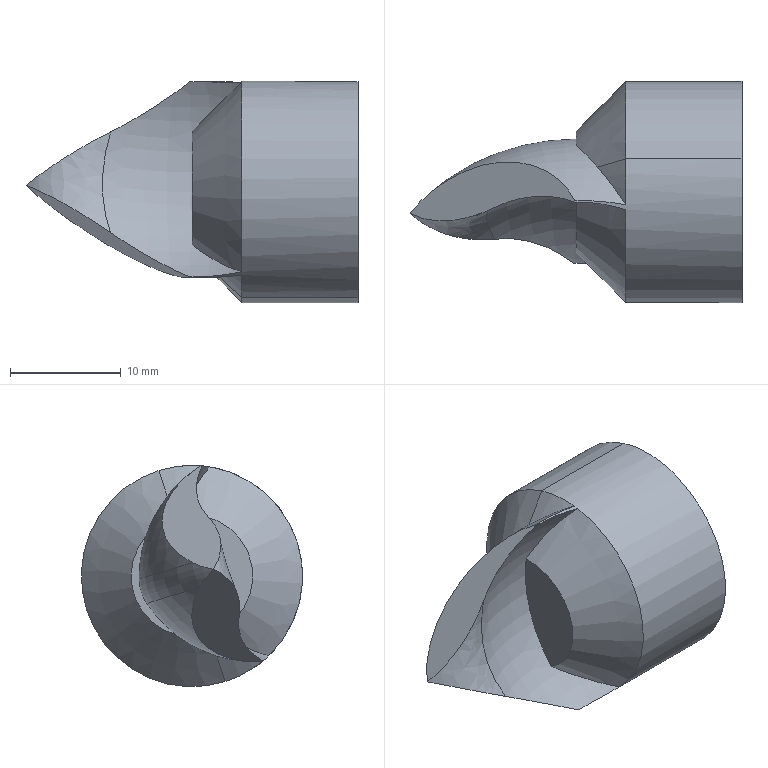Component | SolidWorks | 4-1 | 1 solid | 16 faces | box 30 x 20 x 20 mm | volume 4792 mm3 | plane 5 | cone 4 | torus 4 | cylinder 2 | spline 1 | commonest cylinder face diameters 20 x2
STEP:
#1=CARTESIAN_POINT('',(-2.41,0.4236,0.2806));
#2=VERTEX_POINT('',#1);
#3=CARTESIAN_POINT('',(-2.487,0.5008,0.1405));
#4=VERTEX_POINT('',#3);
#5=CARTESIAN_POINT('',(-2.41,0.4236,0.2806));
#6=CARTESIAN_POINT('',(-2.417,0.4319,0.2705));
#7=CARTESIAN_POINT('',(-2.424,0.4399,0.26));
#8=CARTESIAN_POINT('',(-2.438,0.4549,0.2381));
#9=CARTESIAN_POINT('',(-2.444,0.4618,0.2269));
#10=CARTESIAN_POINT('',(-2.464,0.4812,0.1919));
#11=CARTESIAN_POINT('',(-2.476,0.4921,0.1672));
#12=CARTESIAN_POINT('',(-2.487,0.5008,0.1405));
#13=B_SPLINE_CURVE_WITH_KNOTS('',3,(#5,#6,#7,#8,#9,#10,#11,#12),.UNSPECIFIED.,.F.,.F.,(4,2,2,4),(0.005078,0.006198,0.007317,0.009556),.UNSPECIFIED.);
#14=EDGE_CURVE('',#2,#4,#13,.T.);
#15=ORIENTED_EDGE('',*,*,#14,.F.);
#16=CARTESIAN_POINT('',(-2.31,0.4533,0.3758));
#17=VERTEX_POINT('',#16);
#18=CARTESIAN_POINT('',(-2.487,0.4005,0.2067));
#19=DIRECTION('',(0.7071,0.2108,0.675));
#20=VECTOR('',#19,39.37);
#21=LINE('',#18,#20);
#22=EDGE_CURVE('',#2,#17,#21,.T.);
#23=ORIENTED_EDGE('',*,*,#22,.T.);
#24=CARTESIAN_POINT('',(-2.31,0.2186,-0.3758));
#25=VERTEX_POINT('',#24);
#26=CARTESIAN_POINT('',(-2.31,0.336,0.));
#27=DIRECTION('',(1.,-0.,0.));
#28=DIRECTION('',(0.,0.2981,0.9545));
#29=AXIS2_PLACEMENT_3D('',#26,#27,#28);
#30=CIRCLE('',#29,0.3937);
#31=EDGE_CURVE('',#25,#17,#30,.T.);
#32=ORIENTED_EDGE('',*,*,#31,.F.);
#33=CARTESIAN_POINT('',(-2.41,0.2484,-0.2806));
#34=VERTEX_POINT('',#33);
#35=CARTESIAN_POINT('',(-2.487,0.2714,-0.2067));
#36=DIRECTION('',(0.7071,-0.2108,-0.675));
#37=VECTOR('',#36,39.37);
#38=LINE('',#35,#37);
#39=EDGE_CURVE('',#34,#25,#38,.T.);
#40=ORIENTED_EDGE('',*,*,#39,.F.);
#41=CARTESIAN_POINT('',(-2.487,0.3915,-0.2093));
#42=VERTEX_POINT('',#41);
#43=CARTESIAN_POINT('',(-2.487,0.3915,-0.2093));
#44=CARTESIAN_POINT('',(-2.476,0.3692,-0.2263));
#45=CARTESIAN_POINT('',(-2.464,0.3461,-0.2405));
#46=CARTESIAN_POINT('',(-2.444,0.3104,-0.2581));
#47=CARTESIAN_POINT('',(-2.438,0.2983,-0.2634));
#48=CARTESIAN_POINT('',(-2.424,0.2736,-0.2729));
#49=CARTESIAN_POINT('',(-2.417,0.261,-0.277));
#50=CARTESIAN_POINT('',(-2.41,0.2484,-0.2806));
#51=B_SPLINE_CURVE_WITH_KNOTS('',3,(#43,#44,#45,#46,#47,#48,#49,#50),.UNSPECIFIED.,.F.,.F.,(4,2,2,4),(0.,0.002257,0.003386,0.004515),.UNSPECIFIED.);
#52=EDGE_CURVE('',#42,#34,#51,.T.);
#53=ORIENTED_EDGE('',*,*,#52,.F.);
#54=CARTESIAN_POINT('',(-2.487,0.336,0.));
#55=DIRECTION('',(-1.,0.,-0.));
#56=DIRECTION('',(0.,0.2981,0.9545));
#57=AXIS2_PLACEMENT_3D('',#54,#55,#56);
#58=CIRCLE('',#57,0.2165);
#59=EDGE_CURVE('',#4,#42,#58,.T.);
#60=ORIENTED_EDGE('',*,*,#59,.F.);
#61=EDGE_LOOP('',(#15,#23,#32,#40,#53,#60));
#62=FACE_OUTER_BOUND('',#61,.T.);
#63=CARTESIAN_POINT('',(-2.487,0.336,0.));
#64=DIRECTION('',(1.,-0.,0.));
#65=DIRECTION('',(0.,-0.2981,-0.9545));
#66=AXIS2_PLACEMENT_3D('',#63,#64,#65);
#67=CONICAL_SURFACE('',#66,0.2165,0.7854);
#68=ADVANCED_FACE('',(#62),#67,.T.);
#69=CARTESIAN_POINT('',(-2.31,0.07564,-0.2953));
#70=VERTEX_POINT('',#69);
#71=CARTESIAN_POINT('',(-2.41,0.2484,-0.2806));
#72=CARTESIAN_POINT('',(-2.394,0.2199,-0.2885));
#73=CARTESIAN_POINT('',(-2.377,0.1912,-0.2934));
#74=CARTESIAN_POINT('',(-2.344,0.1335,-0.2981));
#75=CARTESIAN_POINT('',(-2.327,0.1046,-0.2978));
#76=CARTESIAN_POINT('',(-2.31,0.07564,-0.2953));
#77=B_SPLINE_CURVE_WITH_KNOTS('',3,(#71,#72,#73,#74,#75,#76),.UNSPECIFIED.,.F.,.F.,(4,2,4),(0.004515,0.007068,0.009621),.UNSPECIFIED.);
#78=EDGE_CURVE('',#34,#70,#77,.T.);
#79=ORIENTED_EDGE('',*,*,#78,.F.);
#80=ORIENTED_EDGE('',*,*,#39,.T.);
#81=CARTESIAN_POINT('',(-2.31,0.336,0.));
#82=DIRECTION('',(1.,-0.,0.));
#83=DIRECTION('',(0.,0.2981,0.9545));
#84=AXIS2_PLACEMENT_3D('',#81,#82,#83);
#85=CIRCLE('',#84,0.3937);
#86=EDGE_CURVE('',#70,#25,#85,.T.);
#87=ORIENTED_EDGE('',*,*,#86,.F.);
#88=EDGE_LOOP('',(#79,#80,#87));
#89=FACE_OUTER_BOUND('',#88,.T.);
#90=CARTESIAN_POINT('',(-2.487,0.336,0.));
#91=DIRECTION('',(1.,-0.,0.));
#92=DIRECTION('',(0.,-0.2981,-0.9545));
#93=AXIS2_PLACEMENT_3D('',#90,#91,#92);
#94=CONICAL_SURFACE('',#93,0.2165,0.7854);
#95=ADVANCED_FACE('',(#89),#94,.T.);
#96=ORIENTED_EDGE('',*,*,#31,.T.);
#97=CARTESIAN_POINT('',(-1.896,0.4533,0.3758));
#98=VERTEX_POINT('',#97);
#99=CARTESIAN_POINT('',(-2.487,0.4533,0.3758));
#100=DIRECTION('',(1.,-0.,0.));
#101=VECTOR('',#100,39.37);
#102=LINE('',#99,#101);
#103=EDGE_CURVE('',#17,#98,#102,.T.);
#104=ORIENTED_EDGE('',*,*,#103,.T.);
#105=CARTESIAN_POINT('',(-1.896,0.2186,-0.3758));
#106=VERTEX_POINT('',#105);
#107=CARTESIAN_POINT('',(-1.896,0.336,0.));
#108=DIRECTION('',(1.,-0.,0.));
#109=DIRECTION('',(0.,-0.2981,-0.9545));
#110=AXIS2_PLACEMENT_3D('',#107,#108,#109);
#111=CIRCLE('',#110,0.3937);
#112=EDGE_CURVE('',#106,#98,#111,.T.);
#113=ORIENTED_EDGE('',*,*,#112,.F.);
#114=CARTESIAN_POINT('',(-2.487,0.2186,-0.3758));
#115=DIRECTION('',(1.,-0.,0.));
#116=VECTOR('',#115,39.37);
#117=LINE('',#114,#116);
#118=EDGE_CURVE('',#25,#106,#117,.T.);
#119=ORIENTED_EDGE('',*,*,#118,.F.);
#120=EDGE_LOOP('',(#96,#104,#113,#119));
#121=FACE_OUTER_BOUND('',#120,.T.);
#122=CARTESIAN_POINT('',(-2.487,0.336,0.));
#123=DIRECTION('',(1.,-0.,0.));
#124=DIRECTION('',(0.,-0.2981,-0.9545));
#125=AXIS2_PLACEMENT_3D('',#122,#123,#124);
#126=CYLINDRICAL_SURFACE('',#125,0.3937);
#127=ADVANCED_FACE('',(#121),#126,.T.);
#128=CARTESIAN_POINT('',(-2.487,0.524,-0.01135));
#129=VERTEX_POINT('',#128);
#130=CARTESIAN_POINT('',(-2.487,0.05157,-0.005894));
#131=DIRECTION('',(-1.,0.,-0.));
#132=DIRECTION('',(0.,0.2981,0.9545));
#133=AXIS2_PLACEMENT_3D('',#130,#131,#132);
#134=CIRCLE('',#133,0.4724);
#135=EDGE_CURVE('',#4,#129,#134,.T.);
#136=ORIENTED_EDGE('',*,*,#135,.F.);
#137=ORIENTED_EDGE('',*,*,#59,.T.);
#138=CARTESIAN_POINT('',(-2.487,0.497,-0.09765));
#139=VERTEX_POINT('',#138);
#140=CARTESIAN_POINT('',(-2.487,0.1055,0.1667));
#141=DIRECTION('',(-1.,0.,-0.));
#142=DIRECTION('',(0.,-0.2981,-0.9545));
#143=AXIS2_PLACEMENT_3D('',#140,#141,#142);
#144=CIRCLE('',#143,0.4724);
#145=EDGE_CURVE('',#139,#42,#144,.T.);
#146=ORIENTED_EDGE('',*,*,#145,.F.);
#147=CARTESIAN_POINT('',(-2.487,0.3665,-0.009533));
#148=DIRECTION('',(-1.,0.,-0.));
#149=DIRECTION('',(0.,0.2981,0.9545));
#150=AXIS2_PLACEMENT_3D('',#147,#148,#149);
#151=CIRCLE('',#150,0.1575);
#152=EDGE_CURVE('',#129,#139,#151,.T.);
#153=ORIENTED_EDGE('',*,*,#152,.F.);
#154=EDGE_LOOP('',(#136,#137,#146,#153));
#155=FACE_OUTER_BOUND('',#154,.T.);
#156=CARTESIAN_POINT('',(-2.487,0.336,0.));
#157=DIRECTION('',(-1.,0.,0.));
#158=DIRECTION('',(0.,0.2981,0.9545));
#159=AXIS2_PLACEMENT_3D('',#156,#157,#158);
#160=PLANE('',#159);
#161=ADVANCED_FACE('',(#155),#160,.T.);
#162=ORIENTED_EDGE('',*,*,#103,.F.);
#163=CARTESIAN_POINT('',(-2.31,0.29,0.391));
#164=VERTEX_POINT('',#163);
#165=CARTESIAN_POINT('',(-2.31,0.336,0.));
#166=DIRECTION('',(1.,-0.,0.));
#167=DIRECTION('',(0.,0.2981,0.9545));
#168=AXIS2_PLACEMENT_3D('',#165,#166,#167);
#169=CIRCLE('',#168,0.3937);
#170=EDGE_CURVE('',#17,#164,#169,.T.);
#171=ORIENTED_EDGE('',*,*,#170,.T.);
#172=CARTESIAN_POINT('',(-2.491,0.3055,0.3925));
#173=VERTEX_POINT('',#172);
#174=CARTESIAN_POINT('',(-2.491,0.3055,0.3925));
#175=CARTESIAN_POINT('',(-2.43,0.3057,0.3925));
#176=CARTESIAN_POINT('',(-2.37,0.3006,0.3923));
#177=CARTESIAN_POINT('',(-2.31,0.29,0.391));
#178=B_SPLINE_CURVE_WITH_KNOTS('',3,(#174,#175,#176,#177),.UNSPECIFIED.,.F.,.F.,(4,4),(0.007847,0.01243),.UNSPECIFIED.);
#179=EDGE_CURVE('',#173,#164,#178,.T.);
#180=ORIENTED_EDGE('',*,*,#179,.F.);
#181=CARTESIAN_POINT('',(-2.495,0.2997,0.392));
#182=VERTEX_POINT('',#181);
#183=CARTESIAN_POINT('',(-2.495,0.2997,0.392));
#184=CARTESIAN_POINT('',(-2.494,0.3016,0.3922));
#185=CARTESIAN_POINT('',(-2.492,0.3036,0.3924));
#186=CARTESIAN_POINT('',(-2.491,0.3055,0.3925));
#187=(BOUNDED_CURVE()B_SPLINE_CURVE(3,(#183,#184,#185,#186),.UNSPECIFIED.,.F.,.F.)B_SPLINE_CURVE_WITH_KNOTS((4,4),(5.888,5.903),.UNSPECIFIED.)CURVE()GEOMETRIC_REPRESENTATION_ITEM()RATIONAL_B_SPLINE_CURVE((1.,1.,1.,1.))REPRESENTATION_ITEM(''));
#188=EDGE_CURVE('',#182,#173,#187,.T.);
#189=ORIENTED_EDGE('',*,*,#188,.F.);
#190=CARTESIAN_POINT('',(-2.31,0.2726,0.3886));
#191=VERTEX_POINT('',#190);
#192=CARTESIAN_POINT('',(-2.31,0.2726,0.3886));
#193=CARTESIAN_POINT('',(-2.34,0.2819,0.3901));
#194=CARTESIAN_POINT('',(-2.37,0.2889,0.3909));
#195=CARTESIAN_POINT('',(-2.417,0.2957,0.3916));
#196=CARTESIAN_POINT('',(-2.432,0.2974,0.3918));
#197=CARTESIAN_POINT('',(-2.463,0.2995,0.392));
#198=CARTESIAN_POINT('',(-2.479,0.2999,0.392));
#199=CARTESIAN_POINT('',(-2.495,0.2997,0.392));
#200=B_SPLINE_CURVE_WITH_KNOTS('',3,(#192,#193,#194,#195,#196,#197,#198,#199),.UNSPECIFIED.,.F.,.F.,(4,2,2,4),(-0.004538,-0.002172,-0.000989,0.000194),.UNSPECIFIED.);
#201=EDGE_CURVE('',#191,#182,#200,.T.);
#202=ORIENTED_EDGE('',*,*,#201,.F.);
#203=CARTESIAN_POINT('',(-2.31,0.06273,-0.2834));
#204=VERTEX_POINT('',#203);
#205=CARTESIAN_POINT('',(-2.31,0.336,0.));
#206=DIRECTION('',(1.,-0.,0.));
#207=DIRECTION('',(0.,0.2981,0.9545));
#208=AXIS2_PLACEMENT_3D('',#205,#206,#207);
#209=CIRCLE('',#208,0.3937);
#210=EDGE_CURVE('',#191,#204,#209,.T.);
#211=ORIENTED_EDGE('',*,*,#210,.T.);
#212=CARTESIAN_POINT('',(-2.495,0.08307,-0.3017));
#213=VERTEX_POINT('',#212);
#214=CARTESIAN_POINT('',(-2.495,0.08307,-0.3017));
#215=CARTESIAN_POINT('',(-2.479,0.08323,-0.3019));
#216=CARTESIAN_POINT('',(-2.463,0.0829,-0.3016));
#217=CARTESIAN_POINT('',(-2.432,0.08128,-0.3002));
#218=CARTESIAN_POINT('',(-2.417,0.07999,-0.2991));
#219=CARTESIAN_POINT('',(-2.37,0.07479,-0.2946));
#220=CARTESIAN_POINT('',(-2.34,0.06952,-0.29));
#221=CARTESIAN_POINT('',(-2.31,0.06273,-0.2834));
#222=B_SPLINE_CURVE_WITH_KNOTS('',3,(#214,#215,#216,#217,#218,#219,#220,#221),.UNSPECIFIED.,.F.,.F.,(4,2,2,4),(0.004983,0.006166,0.007349,0.009715),.UNSPECIFIED.);
#223=EDGE_CURVE('',#213,#204,#222,.T.);
#224=ORIENTED_EDGE('',*,*,#223,.F.);
#225=CARTESIAN_POINT('',(-2.491,0.08751,-0.3054));
#226=VERTEX_POINT('',#225);
#227=CARTESIAN_POINT('',(-2.491,0.08751,-0.3054));
#228=CARTESIAN_POINT('',(-2.492,0.08602,-0.3042));
#229=CARTESIAN_POINT('',(-2.494,0.08454,-0.303));
#230=CARTESIAN_POINT('',(-2.495,0.08307,-0.3017));
#231=(BOUNDED_CURVE()B_SPLINE_CURVE(3,(#227,#228,#229,#230),.UNSPECIFIED.,.F.,.F.)B_SPLINE_CURVE_WITH_KNOTS((4,4),(0.3803,0.3949),.UNSPECIFIED.)CURVE()GEOMETRIC_REPRESENTATION_ITEM()RATIONAL_B_SPLINE_CURVE((1.,1.,1.,1.))REPRESENTATION_ITEM(''));
#232=EDGE_CURVE('',#226,#213,#231,.T.);
#233=ORIENTED_EDGE('',*,*,#232,.F.);
#234=CARTESIAN_POINT('',(-2.31,0.07564,-0.2953));
#235=CARTESIAN_POINT('',(-2.37,0.08369,-0.3024));
#236=CARTESIAN_POINT('',(-2.43,0.0877,-0.3055));
#237=CARTESIAN_POINT('',(-2.491,0.08751,-0.3054));
#238=B_SPLINE_CURVE_WITH_KNOTS('',3,(#234,#235,#236,#237),.UNSPECIFIED.,.F.,.F.,(4,4),(-0.004494,0.0001071),.UNSPECIFIED.);
#239=EDGE_CURVE('',#70,#226,#238,.T.);
#240=ORIENTED_EDGE('',*,*,#239,.F.);
#241=ORIENTED_EDGE('',*,*,#86,.T.);
#242=ORIENTED_EDGE('',*,*,#118,.T.);
#243=CARTESIAN_POINT('',(-1.896,0.336,0.));
#244=DIRECTION('',(1.,-0.,0.));
#245=DIRECTION('',(0.,-0.2981,-0.9545));
#246=AXIS2_PLACEMENT_3D('',#243,#244,#245);
#247=CIRCLE('',#246,0.3937);
#248=EDGE_CURVE('',#98,#106,#247,.T.);
#249=ORIENTED_EDGE('',*,*,#248,.F.);
#250=EDGE_LOOP('',(#162,#171,#180,#189,#202,#211,#224,#233,#240,#241,#242,#249));
#251=FACE_OUTER_BOUND('',#250,.T.);
#252=CARTESIAN_POINT('',(-2.487,0.336,0.));
#253=DIRECTION('',(1.,-0.,0.));
#254=DIRECTION('',(0.,-0.2981,-0.9545));
#255=AXIS2_PLACEMENT_3D('',#252,#253,#254);
#256=CYLINDRICAL_SURFACE('',#255,0.3937);
#257=ADVANCED_FACE('',(#251),#256,.T.);
#258=CARTESIAN_POINT('',(-2.487,0.2292,-0.1884));
#259=VERTEX_POINT('',#258);
#260=CARTESIAN_POINT('',(-2.487,0.3553,0.2157));
#261=VERTEX_POINT('',#260);
#262=CARTESIAN_POINT('',(-2.487,-0.1526,0.1526));
#263=DIRECTION('',(1.,-0.,0.));
#264=DIRECTION('',(0.,-0.2981,-0.9545));
#265=AXIS2_PLACEMENT_3D('',#262,#263,#264);
#266=CIRCLE('',#265,0.5118);
#267=EDGE_CURVE('',#259,#261,#266,.T.);
#268=ORIENTED_EDGE('',*,*,#267,.F.);
#269=CARTESIAN_POINT('',(-2.487,0.336,0.));
#270=DIRECTION('',(-1.,0.,-0.));
#271=DIRECTION('',(0.,0.2981,0.9545));
#272=AXIS2_PLACEMENT_3D('',#269,#270,#271);
#273=CIRCLE('',#272,0.2165);
#274=EDGE_CURVE('',#259,#261,#273,.T.);
#275=ORIENTED_EDGE('',*,*,#274,.T.);
#276=EDGE_LOOP('',(#268,#275));
#277=FACE_OUTER_BOUND('',#276,.T.);
#278=CARTESIAN_POINT('',(-2.487,0.336,0.));
#279=DIRECTION('',(-1.,0.,0.));
#280=DIRECTION('',(0.,0.2981,0.9545));
#281=AXIS2_PLACEMENT_3D('',#278,#279,#280);
#282=PLANE('',#281);
#283=ADVANCED_FACE('',(#277),#282,.T.);
#284=ORIENTED_EDGE('',*,*,#145,.T.);
#285=ORIENTED_EDGE('',*,*,#52,.T.);
#286=ORIENTED_EDGE('',*,*,#78,.T.);
#287=ORIENTED_EDGE('',*,*,#239,.T.);
#288=CARTESIAN_POINT('',(-3.005,0.3076,-0.03851));
#289=VERTEX_POINT('',#288);
#290=CARTESIAN_POINT('',(-2.491,0.08751,-0.3054));
#291=CARTESIAN_POINT('',(-2.497,0.1007,-0.3059));
#292=CARTESIAN_POINT('',(-2.503,0.1136,-0.3058));
#293=CARTESIAN_POINT('',(-2.517,0.1388,-0.3044));
#294=CARTESIAN_POINT('',(-2.525,0.1509,-0.3032));
#295=CARTESIAN_POINT('',(-2.541,0.1741,-0.2997));
#296=CARTESIAN_POINT('',(-2.55,0.1852,-0.2974));
#297=CARTESIAN_POINT('',(-2.569,0.2065,-0.2919));
#298=CARTESIAN_POINT('',(-2.579,0.2167,-0.2887));
#299=CARTESIAN_POINT('',(-2.609,0.2452,-0.2778));
#300=CARTESIAN_POINT('',(-2.631,0.2618,-0.2688));
#301=CARTESIAN_POINT('',(-2.676,0.2905,-0.248));
#302=CARTESIAN_POINT('',(-2.7,0.3022,-0.2363));
#303=CARTESIAN_POINT('',(-2.748,0.3207,-0.2109));
#304=CARTESIAN_POINT('',(-2.772,0.3275,-0.197));
#305=CARTESIAN_POINT('',(-2.821,0.336,-0.1679));
#306=CARTESIAN_POINT('',(-2.845,0.3379,-0.1527));
#307=CARTESIAN_POINT('',(-2.881,0.3371,-0.129));
#308=CARTESIAN_POINT('',(-2.893,0.3363,-0.1209));
#309=CARTESIAN_POINT('',(-2.916,0.3334,-0.1047));
#310=CARTESIAN_POINT('',(-2.928,0.3315,-0.09653));
#311=CARTESIAN_POINT('',(-2.962,0.324,-0.0719));
#312=CARTESIAN_POINT('',(-2.984,0.3168,-0.05529));
#313=CARTESIAN_POINT('',(-3.005,0.3076,-0.03851));
#314=B_SPLINE_CURVE_WITH_KNOTS('',3,(#290,#291,#292,#293,#294,#295,#296,#297,#298,#299,#300,#301,#302,#303,#304,#305,#306,#307,#308,#309,#310,#311,#312,#313),.UNSPECIFIED.,.F.,.F.,(4,2,2,2,2,2,2,2,2,2,2,4),(0.001469,0.002558,0.003647,0.004736,0.005825,0.008003,0.01018,0.01236,0.01454,0.01563,0.01672,0.01889),.UNSPECIFIED.);
#315=EDGE_CURVE('',#226,#289,#314,.T.);
#316=ORIENTED_EDGE('',*,*,#315,.T.);
#317=CARTESIAN_POINT('',(-2.487,-0.2439,0.1338));
#318=DIRECTION('',(-0.,-0.2981,-0.9545));
#319=DIRECTION('',(-1.,0.,0.));
#320=AXIS2_PLACEMENT_3D('',#317,#318,#319);
#321=CIRCLE('',#320,0.7762);
#322=EDGE_CURVE('',#289,#139,#321,.T.);
#323=ORIENTED_EDGE('',*,*,#322,.T.);
#324=EDGE_LOOP('',(#284,#285,#286,#287,#316,#323));
#325=FACE_OUTER_BOUND('',#324,.T.);
#326=CARTESIAN_POINT('',(-2.487,-0.2035,0.2632));
#327=DIRECTION('',(-0.,-0.2981,-0.9545));
#328=DIRECTION('',(-1.,0.,-0.));
#329=AXIS2_PLACEMENT_3D('',#326,#327,#328);
#330=TOROIDAL_SURFACE('',#329,0.3237,0.4724);
#331=ADVANCED_FACE('',(#325),#330,.T.);
#332=CARTESIAN_POINT('',(-3.078,0.26,0.02359));
#333=VERTEX_POINT('',#332);
#334=CARTESIAN_POINT('',(-3.005,0.3076,-0.03851));
#335=CARTESIAN_POINT('',(-3.032,0.2961,-0.01748));
#336=CARTESIAN_POINT('',(-3.056,0.2798,0.003191));
#337=CARTESIAN_POINT('',(-3.078,0.26,0.02359));
#338=B_SPLINE_CURVE_WITH_KNOTS('',3,(#334,#335,#336,#337),.UNSPECIFIED.,.F.,.F.,(4,4),(0.00000043,0.002707),.UNSPECIFIED.);
#339=EDGE_CURVE('',#289,#333,#338,.T.);
#340=ORIENTED_EDGE('',*,*,#339,.T.);
#341=CARTESIAN_POINT('',(-3.078,0.2601,0.02385));
#342=VERTEX_POINT('',#341);
#343=CARTESIAN_POINT('',(-3.078,0.26,0.02359));
#344=CARTESIAN_POINT('',(-3.078,0.26,0.02368));
#345=CARTESIAN_POINT('',(-3.078,0.26,0.02376));
#346=CARTESIAN_POINT('',(-3.078,0.2601,0.02385));
#347=B_SPLINE_CURVE_WITH_KNOTS('',3,(#343,#344,#345,#346),.UNSPECIFIED.,.F.,.F.,(4,4),(0.,0.00000679),.UNSPECIFIED.);
#348=EDGE_CURVE('',#333,#342,#347,.T.);
#349=ORIENTED_EDGE('',*,*,#348,.T.);
#350=CARTESIAN_POINT('',(-3.005,0.3346,0.04779));
#351=VERTEX_POINT('',#350);
#352=CARTESIAN_POINT('',(-3.078,0.2601,0.02385));
#353=CARTESIAN_POINT('',(-3.056,0.288,0.02934));
#354=CARTESIAN_POINT('',(-3.032,0.3132,0.03705));
#355=CARTESIAN_POINT('',(-3.005,0.3346,0.04779));
#356=B_SPLINE_CURVE_WITH_KNOTS('',3,(#352,#353,#354,#355),.UNSPECIFIED.,.F.,.F.,(4,4),(0.00000922,0.002716),.UNSPECIFIED.);
#357=EDGE_CURVE('',#342,#351,#356,.T.);
#358=ORIENTED_EDGE('',*,*,#357,.T.);
#359=CARTESIAN_POINT('',(-2.487,-0.217,0.2201));
#360=DIRECTION('',(-0.,-0.2981,-0.9545));
#361=DIRECTION('',(-1.,0.,0.));
#362=AXIS2_PLACEMENT_3D('',#359,#360,#361);
#363=CIRCLE('',#362,0.7762);
#364=EDGE_CURVE('',#351,#129,#363,.T.);
#365=ORIENTED_EDGE('',*,*,#364,.T.);
#366=ORIENTED_EDGE('',*,*,#152,.T.);
#367=ORIENTED_EDGE('',*,*,#322,.F.);
#368=EDGE_LOOP('',(#340,#349,#358,#365,#366,#367));
#369=FACE_OUTER_BOUND('',#368,.T.);
#370=CARTESIAN_POINT('',(-2.487,-0.2305,0.1769));
#371=DIRECTION('',(-0.,-0.2981,-0.9545));
#372=DIRECTION('',(-1.,0.,-0.));
#373=AXIS2_PLACEMENT_3D('',#370,#371,#372);
#374=TOROIDAL_SURFACE('',#373,0.6254,0.1575);
#375=ADVANCED_FACE('',(#369),#374,.T.);
#376=CARTESIAN_POINT('',(-3.005,0.3346,0.04779));
#377=CARTESIAN_POINT('',(-2.984,0.3517,0.05638));
#378=CARTESIAN_POINT('',(-2.962,0.3671,0.066));
#379=CARTESIAN_POINT('',(-2.928,0.3873,0.08202));
#380=CARTESIAN_POINT('',(-2.916,0.3936,0.08763));
#381=CARTESIAN_POINT('',(-2.893,0.4051,0.0994));
#382=CARTESIAN_POINT('',(-2.881,0.4105,0.1056));
#383=CARTESIAN_POINT('',(-2.845,0.4246,0.1247));
#384=CARTESIAN_POINT('',(-2.82,0.4316,0.1382));
#385=CARTESIAN_POINT('',(-2.784,0.4387,0.1597));
#386=CARTESIAN_POINT('',(-2.772,0.4405,0.167));
#387=CARTESIAN_POINT('',(-2.748,0.4427,0.1821));
#388=CARTESIAN_POINT('',(-2.736,0.4432,0.19));
#389=CARTESIAN_POINT('',(-2.699,0.4427,0.2137));
#390=CARTESIAN_POINT('',(-2.676,0.4397,0.2299));
#391=CARTESIAN_POINT('',(-2.642,0.431,0.2546));
#392=CARTESIAN_POINT('',(-2.631,0.4274,0.263));
#393=CARTESIAN_POINT('',(-2.61,0.4188,0.2798));
#394=CARTESIAN_POINT('',(-2.599,0.4137,0.2883));
#395=CARTESIAN_POINT('',(-2.569,0.3964,0.3137));
#396=CARTESIAN_POINT('',(-2.55,0.3822,0.3302));
#397=CARTESIAN_POINT('',(-2.525,0.3564,0.3546));
#398=CARTESIAN_POINT('',(-2.517,0.347,0.3626));
#399=CARTESIAN_POINT('',(-2.503,0.3272,0.378));
#400=CARTESIAN_POINT('',(-2.497,0.3166,0.3854));
#401=CARTESIAN_POINT('',(-2.491,0.3055,0.3925));
#402=B_SPLINE_CURVE_WITH_KNOTS('',3,(#376,#377,#378,#379,#380,#381,#382,#383,#384,#385,#386,#387,#388,#389,#390,#391,#392,#393,#394,#395,#396,#397,#398,#399,#400,#401),.UNSPECIFIED.,.F.,.F.,(4,2,2,2,2,2,2,2,2,2,2,2,4),(0.0007613,0.002936,0.004023,0.00511,0.007284,0.008371,0.009459,0.01163,0.01272,0.01381,0.01598,0.01707,0.01816),.UNSPECIFIED.);
#403=EDGE_CURVE('',#351,#173,#402,.T.);
#404=ORIENTED_EDGE('',*,*,#403,.T.);
#405=ORIENTED_EDGE('',*,*,#179,.T.);
#406=CARTESIAN_POINT('',(-2.31,0.29,0.391));
#407=CARTESIAN_POINT('',(-2.327,0.3152,0.3765));
#408=CARTESIAN_POINT('',(-2.344,0.3392,0.3603));
#409=CARTESIAN_POINT('',(-2.377,0.384,0.3236));
#410=CARTESIAN_POINT('',(-2.394,0.4047,0.3033));
#411=CARTESIAN_POINT('',(-2.41,0.4236,0.2806));
#412=B_SPLINE_CURVE_WITH_KNOTS('',3,(#406,#407,#408,#409,#410,#411),.UNSPECIFIED.,.F.,.F.,(4,2,4),(0.,0.002539,0.005078),.UNSPECIFIED.);
#413=EDGE_CURVE('',#164,#2,#412,.T.);
#414=ORIENTED_EDGE('',*,*,#413,.T.);
#415=ORIENTED_EDGE('',*,*,#14,.T.);
#416=ORIENTED_EDGE('',*,*,#135,.T.);
#417=ORIENTED_EDGE('',*,*,#364,.F.);
#418=EDGE_LOOP('',(#404,#405,#414,#415,#416,#417));
#419=FACE_OUTER_BOUND('',#418,.T.);
#420=CARTESIAN_POINT('',(-2.487,-0.2574,0.0906));
#421=DIRECTION('',(-0.,-0.2981,-0.9545));
#422=DIRECTION('',(-1.,0.,-0.));
#423=AXIS2_PLACEMENT_3D('',#420,#421,#422);
#424=TOROIDAL_SURFACE('',#423,0.3237,0.4724);
#425=ADVANCED_FACE('',(#419),#424,.T.);
#426=ORIENTED_EDGE('',*,*,#223,.T.);
#427=CARTESIAN_POINT('',(-2.31,0.06273,-0.2834));
#428=CARTESIAN_POINT('',(-2.338,0.09588,-0.2761));
#429=CARTESIAN_POINT('',(-2.367,0.1267,-0.2642));
#430=CARTESIAN_POINT('',(-2.411,0.1687,-0.2402));
#431=CARTESIAN_POINT('',(-2.426,0.1821,-0.2312));
#432=CARTESIAN_POINT('',(-2.456,0.2071,-0.2111));
#433=CARTESIAN_POINT('',(-2.472,0.2186,-0.2002));
#434=CARTESIAN_POINT('',(-2.487,0.2292,-0.1884));
#435=B_SPLINE_CURVE_WITH_KNOTS('',3,(#427,#428,#429,#430,#431,#432,#433,#434),.UNSPECIFIED.,.F.,.F.,(4,2,2,4),(0.,0.003321,0.004982,0.006643),.UNSPECIFIED.);
#436=EDGE_CURVE('',#204,#259,#435,.T.);
#437=ORIENTED_EDGE('',*,*,#436,.T.);
#438=ORIENTED_EDGE('',*,*,#267,.T.);
#439=CARTESIAN_POINT('',(-2.487,0.3553,0.2157));
#440=CARTESIAN_POINT('',(-2.456,0.3515,0.2471));
#441=CARTESIAN_POINT('',(-2.426,0.3424,0.2776));
#442=CARTESIAN_POINT('',(-2.382,0.3215,0.3212));
#443=CARTESIAN_POINT('',(-2.367,0.3133,0.3355));
#444=CARTESIAN_POINT('',(-2.338,0.2946,0.363));
#445=CARTESIAN_POINT('',(-2.324,0.2841,0.3761));
#446=CARTESIAN_POINT('',(-2.31,0.2726,0.3886));
#447=B_SPLINE_CURVE_WITH_KNOTS('',3,(#439,#440,#441,#442,#443,#444,#445,#446),.UNSPECIFIED.,.F.,.F.,(4,2,2,4),(0.,0.003322,0.004983,0.006644),.UNSPECIFIED.);
#448=EDGE_CURVE('',#261,#191,#447,.T.);
#449=ORIENTED_EDGE('',*,*,#448,.T.);
#450=ORIENTED_EDGE('',*,*,#201,.T.);
#451=CARTESIAN_POINT('',(-2.777,0.2803,0.2138));
#452=VERTEX_POINT('',#451);
#453=CARTESIAN_POINT('',(-2.495,0.2997,0.392));
#454=CARTESIAN_POINT('',(-2.516,0.3083,0.3752));
#455=CARTESIAN_POINT('',(-2.539,0.3143,0.3587));
#456=CARTESIAN_POINT('',(-2.574,0.3195,0.3344));
#457=CARTESIAN_POINT('',(-2.585,0.3206,0.3263));
#458=CARTESIAN_POINT('',(-2.609,0.3215,0.3104));
#459=CARTESIAN_POINT('',(-2.621,0.3213,0.3027));
#460=CARTESIAN_POINT('',(-2.657,0.3187,0.28));
#461=CARTESIAN_POINT('',(-2.681,0.3145,0.2656));
#462=CARTESIAN_POINT('',(-2.718,0.3044,0.2451));
#463=CARTESIAN_POINT('',(-2.73,0.3004,0.2384));
#464=CARTESIAN_POINT('',(-2.754,0.2912,0.2257));
#465=CARTESIAN_POINT('',(-2.765,0.2861,0.2196));
#466=CARTESIAN_POINT('',(-2.777,0.2803,0.2138));
#467=B_SPLINE_CURVE_WITH_KNOTS('',3,(#453,#454,#455,#456,#457,#458,#459,#460,#461,#462,#463,#464,#465,#466),.UNSPECIFIED.,.F.,.F.,(4,2,2,2,2,2,4),(0.0002605,0.00243,0.003515,0.004599,0.006769,0.007853,0.008938),.UNSPECIFIED.);
#468=EDGE_CURVE('',#182,#452,#467,.T.);
#469=ORIENTED_EDGE('',*,*,#468,.T.);
#470=CARTESIAN_POINT('',(-2.777,0.1685,-0.1442));
#471=VERTEX_POINT('',#470);
#472=CARTESIAN_POINT('',(-2.777,0.2803,0.2138));
#473=CARTESIAN_POINT('',(-2.782,0.2797,0.1984));
#474=CARTESIAN_POINT('',(-2.786,0.2785,0.1828));
#475=CARTESIAN_POINT('',(-2.793,0.2751,0.1516));
#476=CARTESIAN_POINT('',(-2.796,0.2729,0.136));
#477=CARTESIAN_POINT('',(-2.803,0.2646,0.08945));
#478=CARTESIAN_POINT('',(-2.806,0.2571,0.05848));
#479=CARTESIAN_POINT('',(-2.806,0.2378,-0.003283));
#480=CARTESIAN_POINT('',(-2.803,0.2264,-0.03302));
#481=CARTESIAN_POINT('',(-2.796,0.2066,-0.07599));
#482=CARTESIAN_POINT('',(-2.793,0.1996,-0.09004));
#483=CARTESIAN_POINT('',(-2.786,0.1847,-0.1176));
#484=CARTESIAN_POINT('',(-2.782,0.1768,-0.1311));
#485=CARTESIAN_POINT('',(-2.777,0.1685,-0.1442));
#486=B_SPLINE_CURVE_WITH_KNOTS('',3,(#472,#473,#474,#475,#476,#477,#478,#479,#480,#481,#482,#483,#484,#485),.UNSPECIFIED.,.F.,.F.,(4,2,2,2,2,2,4),(0.,0.001232,0.002464,0.004929,0.007393,0.008625,0.009857),.UNSPECIFIED.);
#487=EDGE_CURVE('',#452,#471,#486,.T.);
#488=ORIENTED_EDGE('',*,*,#487,.T.);
#489=CARTESIAN_POINT('',(-2.777,0.1685,-0.1442));
#490=CARTESIAN_POINT('',(-2.754,0.1713,-0.1602));
#491=CARTESIAN_POINT('',(-2.73,0.1717,-0.1758));
#492=CARTESIAN_POINT('',(-2.694,0.1684,-0.1984));
#493=CARTESIAN_POINT('',(-2.682,0.1666,-0.2058));
#494=CARTESIAN_POINT('',(-2.657,0.1618,-0.2202));
#495=CARTESIAN_POINT('',(-2.645,0.1588,-0.2271));
#496=CARTESIAN_POINT('',(-2.609,0.148,-0.2472));
#497=CARTESIAN_POINT('',(-2.586,0.1384,-0.2596));
#498=CARTESIAN_POINT('',(-2.551,0.1202,-0.2768));
#499=CARTESIAN_POINT('',(-2.539,0.1136,-0.2822));
#500=CARTESIAN_POINT('',(-2.517,0.09915,-0.2925));
#501=CARTESIAN_POINT('',(-2.506,0.09139,-0.2973));
#502=CARTESIAN_POINT('',(-2.495,0.08307,-0.3017));
#503=B_SPLINE_CURVE_WITH_KNOTS('',3,(#489,#490,#491,#492,#493,#494,#495,#496,#497,#498,#499,#500,#501,#502),.UNSPECIFIED.,.F.,.F.,(4,2,2,2,2,2,4),(0.005374,0.007535,0.008615,0.009695,0.01186,0.01294,0.01402),.UNSPECIFIED.);
#504=EDGE_CURVE('',#471,#213,#503,.T.);
#505=ORIENTED_EDGE('',*,*,#504,.T.);
#506=EDGE_LOOP('',(#426,#437,#438,#449,#450,#469,#488,#505));
#507=FACE_OUTER_BOUND('',#506,.T.);
#508=CARTESIAN_POINT('',(-2.487,-0.2305,0.1769));
#509=DIRECTION('',(-0.,-0.2981,-0.9545));
#510=DIRECTION('',(-1.,0.,0.));
#511=AXIS2_PLACEMENT_3D('',#508,#509,#510);
#512=TOROIDAL_SURFACE('',#511,0.08161,0.5118);
#513=ADVANCED_FACE('',(#507),#512,.F.);
#514=ORIENTED_EDGE('',*,*,#468,.F.);
#515=ORIENTED_EDGE('',*,*,#188,.T.);
#516=ORIENTED_EDGE('',*,*,#403,.F.);
#517=ORIENTED_EDGE('',*,*,#357,.F.);
#518=CARTESIAN_POINT('',(-3.078,0.2601,0.02385));
#519=CARTESIAN_POINT('',(-3.056,0.2478,0.04197));
#520=CARTESIAN_POINT('',(-3.032,0.2404,0.05966));
#521=CARTESIAN_POINT('',(-2.995,0.2345,0.08574));
#522=CARTESIAN_POINT('',(-2.982,0.2335,0.09441));
#523=CARTESIAN_POINT('',(-2.957,0.233,0.1112));
#524=CARTESIAN_POINT('',(-2.944,0.2336,0.1194));
#525=CARTESIAN_POINT('',(-2.905,0.2375,0.1434));
#526=CARTESIAN_POINT('',(-2.88,0.2428,0.1586));
#527=CARTESIAN_POINT('',(-2.841,0.2542,0.1804));
#528=CARTESIAN_POINT('',(-2.828,0.2586,0.1874));
#529=CARTESIAN_POINT('',(-2.802,0.2686,0.201));
#530=CARTESIAN_POINT('',(-2.79,0.2741,0.2076));
#531=CARTESIAN_POINT('',(-2.777,0.2803,0.2138));
#532=B_SPLINE_CURVE_WITH_KNOTS('',3,(#518,#519,#520,#521,#522,#523,#524,#525,#526,#527,#528,#529,#530,#531),.UNSPECIFIED.,.F.,.F.,(4,2,2,2,2,2,4),(-0.007234,-0.0049,-0.003733,-0.002566,-0.0002321,0.000935,0.002102),.UNSPECIFIED.);
#533=EDGE_CURVE('',#342,#452,#532,.T.);
#534=ORIENTED_EDGE('',*,*,#533,.T.);
#535=EDGE_LOOP('',(#514,#515,#516,#517,#534));
#536=FACE_OUTER_BOUND('',#535,.T.);
#537=CARTESIAN_POINT('',(-2.487,-0.1367,0.5334));
#538=DIRECTION('',(0.5289,-0.253,-0.8101));
#539=DIRECTION('',(-0.8487,-0.1577,-0.5048));
#540=AXIS2_PLACEMENT_3D('',#537,#538,#539);
#541=PLANE('',#540);
#542=ADVANCED_FACE('',(#536),#541,.F.);
#543=ORIENTED_EDGE('',*,*,#315,.F.);
#544=ORIENTED_EDGE('',*,*,#232,.T.);
#545=ORIENTED_EDGE('',*,*,#504,.F.);
#546=CARTESIAN_POINT('',(-2.777,0.1685,-0.1442));
#547=CARTESIAN_POINT('',(-2.802,0.1655,-0.1268));
#548=CARTESIAN_POINT('',(-2.828,0.1652,-0.1101));
#549=CARTESIAN_POINT('',(-2.879,0.169,-0.07786));
#550=CARTESIAN_POINT('',(-2.905,0.1732,-0.06234));
#551=CARTESIAN_POINT('',(-2.957,0.1873,-0.03276));
#552=CARTESIAN_POINT('',(-2.982,0.197,-0.01911));
#553=CARTESIAN_POINT('',(-3.019,0.2166,-0.0009509));
#554=CARTESIAN_POINT('',(-3.032,0.224,0.004751));
#555=CARTESIAN_POINT('',(-3.055,0.2406,0.01505));
#556=CARTESIAN_POINT('',(-3.067,0.2498,0.01964));
#557=CARTESIAN_POINT('',(-3.078,0.26,0.02359));
#558=B_SPLINE_CURVE_WITH_KNOTS('',3,(#546,#547,#548,#549,#550,#551,#552,#553,#554,#555,#556,#557),.UNSPECIFIED.,.F.,.F.,(4,2,2,2,2,4),(0.,0.002309,0.004618,0.006927,0.008082,0.009236),.UNSPECIFIED.);
#559=EDGE_CURVE('',#471,#333,#558,.T.);
#560=ORIENTED_EDGE('',*,*,#559,.T.);
#561=ORIENTED_EDGE('',*,*,#339,.F.);
#562=EDGE_LOOP('',(#543,#544,#545,#560,#561));
#563=FACE_OUTER_BOUND('',#562,.T.);
#564=CARTESIAN_POINT('',(-2.487,-0.3563,-0.1696));
#565=DIRECTION('',(0.5289,0.253,0.8101));
#566=DIRECTION('',(0.8487,-0.1577,-0.5048));
#567=AXIS2_PLACEMENT_3D('',#564,#565,#566);
#568=PLANE('',#567);
#569=ADVANCED_FACE('',(#563),#568,.F.);
#570=ORIENTED_EDGE('',*,*,#559,.F.);
#571=ORIENTED_EDGE('',*,*,#487,.F.);
#572=ORIENTED_EDGE('',*,*,#533,.F.);
#573=ORIENTED_EDGE('',*,*,#348,.F.);
#574=EDGE_LOOP('',(#570,#571,#572,#573));
#575=FACE_OUTER_BOUND('',#574,.T.);
#576=CARTESIAN_POINT('',(-2.776,0.1673,-0.146));
#577=CARTESIAN_POINT('',(-2.915,0.07294,-0.1358));
#578=CARTESIAN_POINT('',(-3.038,0.1453,-0.2265));
#579=CARTESIAN_POINT('',(-2.781,0.1757,-0.133));
#580=CARTESIAN_POINT('',(-2.921,0.08218,-0.1215));
#581=CARTESIAN_POINT('',(-3.044,0.1573,-0.2077));
#582=CARTESIAN_POINT('',(-2.785,0.1838,-0.1193));
#583=CARTESIAN_POINT('',(-2.925,0.09112,-0.1065));
#584=CARTESIAN_POINT('',(-3.05,0.169,-0.188));
#585=CARTESIAN_POINT('',(-2.793,0.1989,-0.09142));
#586=CARTESIAN_POINT('',(-2.933,0.1079,-0.07605));
#587=CARTESIAN_POINT('',(-3.061,0.191,-0.148));
#588=CARTESIAN_POINT('',(-2.796,0.2061,-0.07721));
#589=CARTESIAN_POINT('',(-2.937,0.1158,-0.06048));
#590=CARTESIAN_POINT('',(-3.065,0.2013,-0.1275));
#591=CARTESIAN_POINT('',(-2.803,0.2261,-0.03374));
#592=CARTESIAN_POINT('',(-2.945,0.1379,-0.01283));
#593=CARTESIAN_POINT('',(-3.076,0.2302,-0.06496));
#594=CARTESIAN_POINT('',(-2.806,0.2377,-0.003652));
#595=CARTESIAN_POINT('',(-2.947,0.1507,0.02019));
#596=CARTESIAN_POINT('',(-3.079,0.247,-0.02165));
#597=CARTESIAN_POINT('',(-2.806,0.2572,0.05886));
#598=CARTESIAN_POINT('',(-2.947,0.1721,0.0888));
#599=CARTESIAN_POINT('',(-3.079,0.2751,0.06836));
#600=CARTESIAN_POINT('',(-2.803,0.2648,0.09022));
#601=CARTESIAN_POINT('',(-2.945,0.1804,0.1232));
#602=CARTESIAN_POINT('',(-3.076,0.286,0.1135));
#603=CARTESIAN_POINT('',(-2.796,0.2731,0.1374));
#604=CARTESIAN_POINT('',(-2.937,0.1893,0.175));
#605=CARTESIAN_POINT('',(-3.065,0.2978,0.1815));
#606=CARTESIAN_POINT('',(-2.793,0.2753,0.1532));
#607=CARTESIAN_POINT('',(-2.933,0.1917,0.1923));
#608=CARTESIAN_POINT('',(-3.061,0.3009,0.2042));
#609=CARTESIAN_POINT('',(-2.785,0.2787,0.1847));
#610=CARTESIAN_POINT('',(-2.925,0.1953,0.227));
#611=CARTESIAN_POINT('',(-3.05,0.3057,0.2496));
#612=CARTESIAN_POINT('',(-2.781,0.2798,0.2006));
#613=CARTESIAN_POINT('',(-2.921,0.1964,0.2444));
#614=CARTESIAN_POINT('',(-3.044,0.3073,0.2725));
#615=CARTESIAN_POINT('',(-2.776,0.2804,0.216));
#616=CARTESIAN_POINT('',(-2.915,0.197,0.2614));
#617=CARTESIAN_POINT('',(-3.038,0.3081,0.2948));
#618=(BOUNDED_SURFACE()B_SPLINE_SURFACE(3,2,((#576,#577,#578),(#579,#580,#581),(#582,#583,#584),(#585,#586,#587),(#588,#589,#590),(#591,#592,#593),(#594,#595,#596),(#597,#598,#599),(#600,#601,#602),(#603,#604,#605),(#606,#607,#608),(#609,#610,#611),(#612,#613,#614),(#615,#616,#617)),.UNSPECIFIED.,.F.,.F.,.T.)B_SPLINE_SURFACE_WITH_KNOTS((4,2,2,2,2,2,4),(3,3),(0.0398,0.0416,0.04339,0.04698,0.05058,0.05237,0.05417),(0.,0.9624),.UNSPECIFIED.)GEOMETRIC_REPRESENTATION_ITEM()RATIONAL_B_SPLINE_SURFACE(((1.,0.8083,0.9856),(1.,0.8084,0.9856),(1.,0.8085,0.9856),(1.,0.8087,0.9856),(1.,0.8087,0.9856),(1.,0.8089,0.9856),(1.,0.8089,0.9856),(1.,0.8089,0.9856),(1.,0.8089,0.9856),(1.,0.8087,0.9856),(1.,0.8087,0.9856),(1.,0.8085,0.9856),(1.,0.8084,0.9856),(1.,0.8083,0.9856)))REPRESENTATION_ITEM('')SURFACE());
#619=ADVANCED_FACE('',(#575),#618,.T.);
#620=ORIENTED_EDGE('',*,*,#436,.F.);
#621=ORIENTED_EDGE('',*,*,#210,.F.);
#622=ORIENTED_EDGE('',*,*,#448,.F.);
#623=ORIENTED_EDGE('',*,*,#274,.F.);
#624=EDGE_LOOP('',(#620,#621,#622,#623));
#625=FACE_OUTER_BOUND('',#624,.T.);
#626=CARTESIAN_POINT('',(-2.487,0.336,0.));
#627=DIRECTION('',(1.,-0.,0.));
#628=DIRECTION('',(0.,-0.2981,-0.9545));
#629=AXIS2_PLACEMENT_3D('',#626,#627,#628);
#630=CONICAL_SURFACE('',#629,0.2165,0.7854);
#631=ADVANCED_FACE('',(#625),#630,.T.);
#632=ORIENTED_EDGE('',*,*,#22,.F.);
#633=ORIENTED_EDGE('',*,*,#413,.F.);
#634=ORIENTED_EDGE('',*,*,#170,.F.);
#635=EDGE_LOOP('',(#632,#633,#634));
#636=FACE_OUTER_BOUND('',#635,.T.);
#637=CARTESIAN_POINT('',(-2.487,0.336,0.));
#638=DIRECTION('',(1.,-0.,0.));
#639=DIRECTION('',(0.,-0.2981,-0.9545));
#640=AXIS2_PLACEMENT_3D('',#637,#638,#639);
#641=CONICAL_SURFACE('',#640,0.2165,0.7854);
#642=ADVANCED_FACE('',(#636),#641,.T.);
#643=ORIENTED_EDGE('',*,*,#112,.T.);
#644=ORIENTED_EDGE('',*,*,#248,.T.);
#645=EDGE_LOOP('',(#643,#644));
#646=FACE_OUTER_BOUND('',#645,.T.);
#647=CARTESIAN_POINT('',(-1.896,0.336,0.));
#648=DIRECTION('',(1.,-0.,0.));
#649=DIRECTION('',(-0.,-0.2981,-0.9545));
#650=AXIS2_PLACEMENT_3D('',#647,#648,#649);
#651=PLANE('',#650);
#652=ADVANCED_FACE('',(#646),#651,.T.);
#653=CLOSED_SHELL('',(#68,#95,#127,#161,#257,#283,#331,#375,#425,#513,#542,#569,#619,#631,#642,#652));
#654=MANIFOLD_SOLID_BREP('',#653);
#655=CARTESIAN_POINT('',(0.,0.,0.));
#656=DIRECTION('',(0.,0.,1.));
#657=DIRECTION('',(1.,0.,0.));
#658=AXIS2_PLACEMENT_3D('',#655,#656,#657);
#659=(LENGTH_UNIT()NAMED_UNIT(*)SI_UNIT($,.METRE.));
#660=LENGTH_MEASURE_WITH_UNIT(LENGTH_MEASURE(0.0254),#659);
#661=DIMENSIONAL_EXPONENTS(1.,0.,0.,0.,0.,0.,0.);
#662=(CONVERSION_BASED_UNIT('',#660)LENGTH_UNIT()NAMED_UNIT(#661));
#663=UNCERTAINTY_MEASURE_WITH_UNIT(LENGTH_MEASURE(0.00001),#662,'','');
#664=(NAMED_UNIT(*)PLANE_ANGLE_UNIT()SI_UNIT($,.RADIAN.));
#665=(NAMED_UNIT(*)SI_UNIT($,.STERADIAN.)SOLID_ANGLE_UNIT());
#666=(GEOMETRIC_REPRESENTATION_CONTEXT(3)GLOBAL_UNCERTAINTY_ASSIGNED_CONTEXT((#663))GLOBAL_UNIT_ASSIGNED_CONTEXT((#662,#664,#665))REPRESENTATION_CONTEXT('',''));
#667=ADVANCED_BREP_SHAPE_REPRESENTATION('',(#654,#658),#666);
#668=COLOUR_RGB('',0.7922,0.8196,0.9333);
#669=FILL_AREA_STYLE_COLOUR('',#668);
#670=FILL_AREA_STYLE('',(#669));
#671=SURFACE_STYLE_FILL_AREA(#670);
#672=SURFACE_SIDE_STYLE('',(#671));
#673=SURFACE_STYLE_USAGE(.BOTH.,#672);
#674=PRESENTATION_STYLE_ASSIGNMENT((#673));
#675=STYLED_ITEM('',(#674),#654);
#676=PRESENTATION_LAYER_ASSIGNMENT('','',(#675));
#677=(LENGTH_UNIT()NAMED_UNIT(*)SI_UNIT($,.METRE.));
#678=LENGTH_MEASURE_WITH_UNIT(LENGTH_MEASURE(0.0254),#677);
#679=DIMENSIONAL_EXPONENTS(1.,0.,0.,0.,0.,0.,0.);
#680=(CONVERSION_BASED_UNIT('',#678)LENGTH_UNIT()NAMED_UNIT(#679));
#681=UNCERTAINTY_MEASURE_WITH_UNIT(LENGTH_MEASURE(0.00001),#680,'','');
#682=(NAMED_UNIT(*)PLANE_ANGLE_UNIT()SI_UNIT($,.RADIAN.));
#683=(NAMED_UNIT(*)SI_UNIT($,.STERADIAN.)SOLID_ANGLE_UNIT());
#684=(GEOMETRIC_REPRESENTATION_CONTEXT(3)GLOBAL_UNCERTAINTY_ASSIGNED_CONTEXT((#681))GLOBAL_UNIT_ASSIGNED_CONTEXT((#680,#682,#683))REPRESENTATION_CONTEXT('',''));
#685=MECHANICAL_DESIGN_GEOMETRIC_PRESENTATION_REPRESENTATION('',(#675),#684);